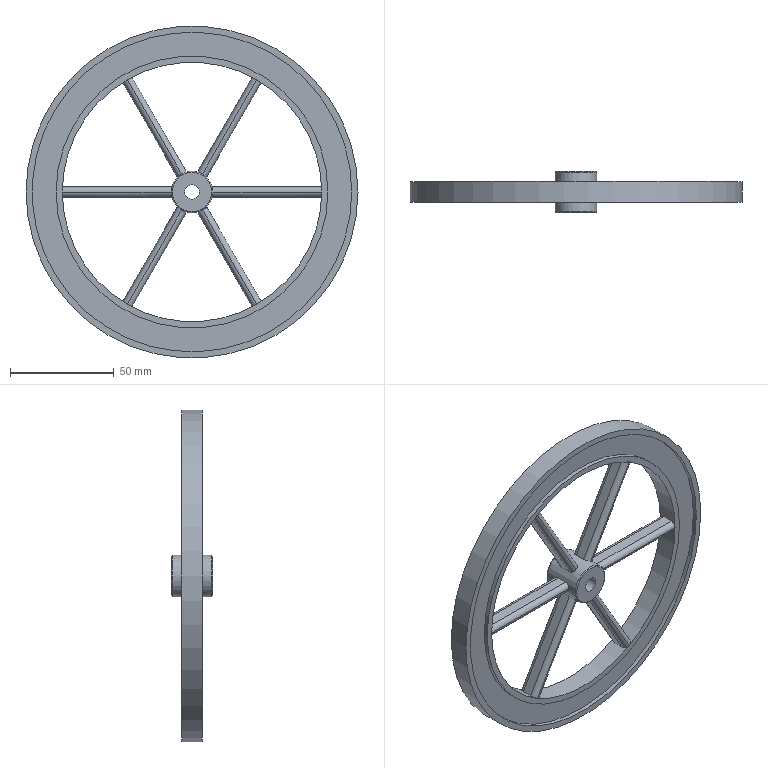Component | NX | FLYWHEEL | 1 solid | 59 faces | volume 77338 mm3 | cylinder 37 | plane 20 | torus 2 | commonest cylinder face diameters 5 x24 125 x6 154 x2 131 x2 160 x1 20 x1 7 x1